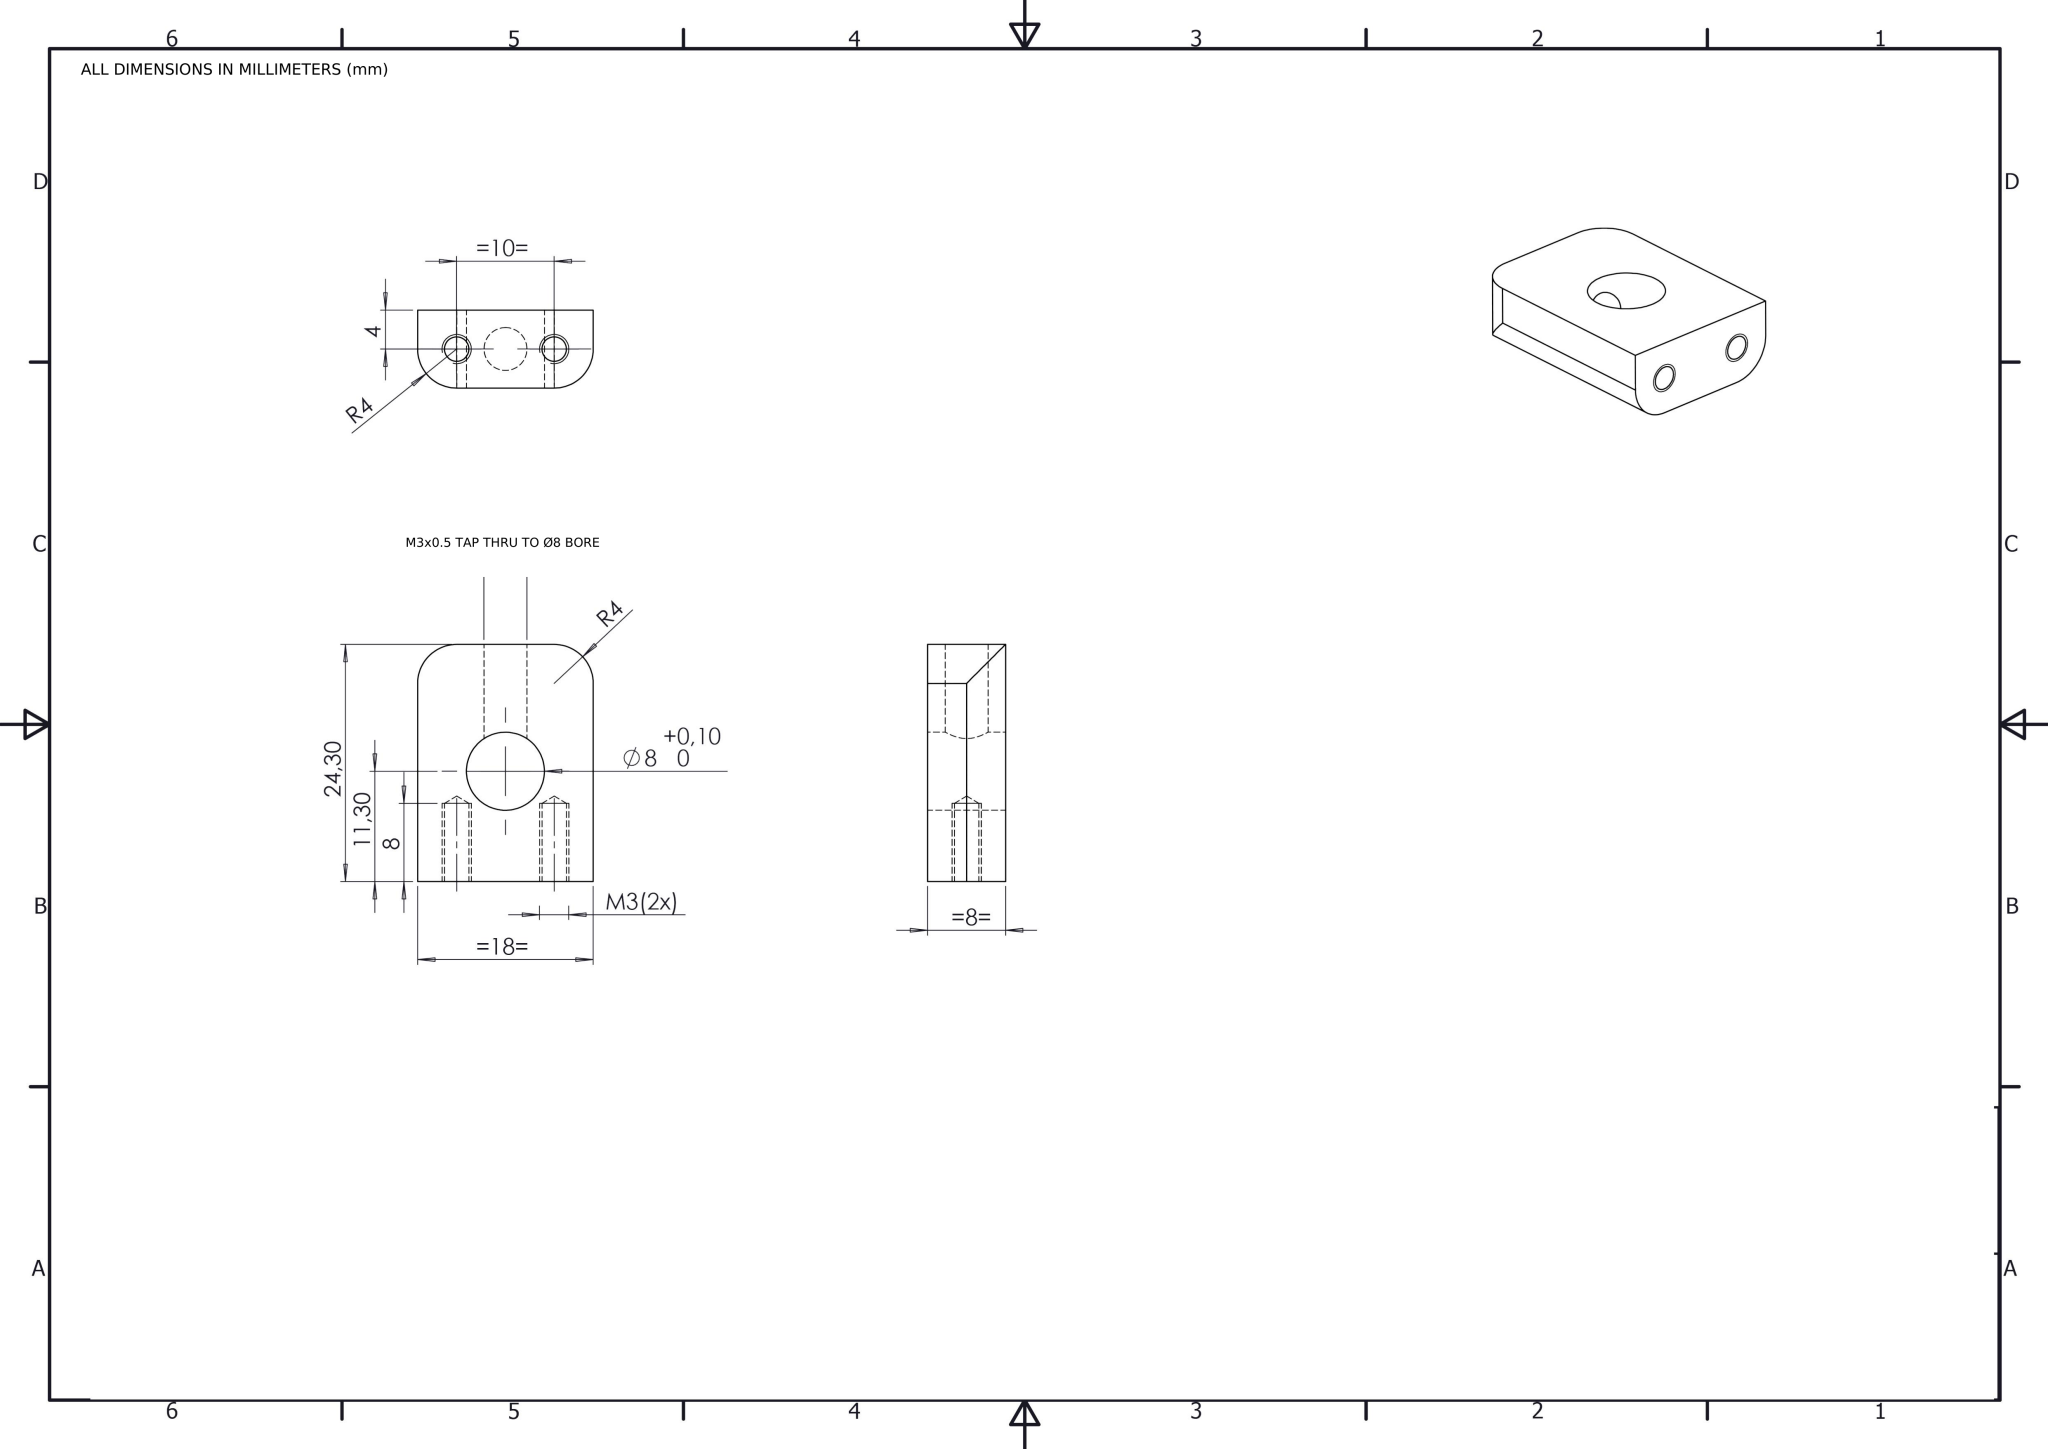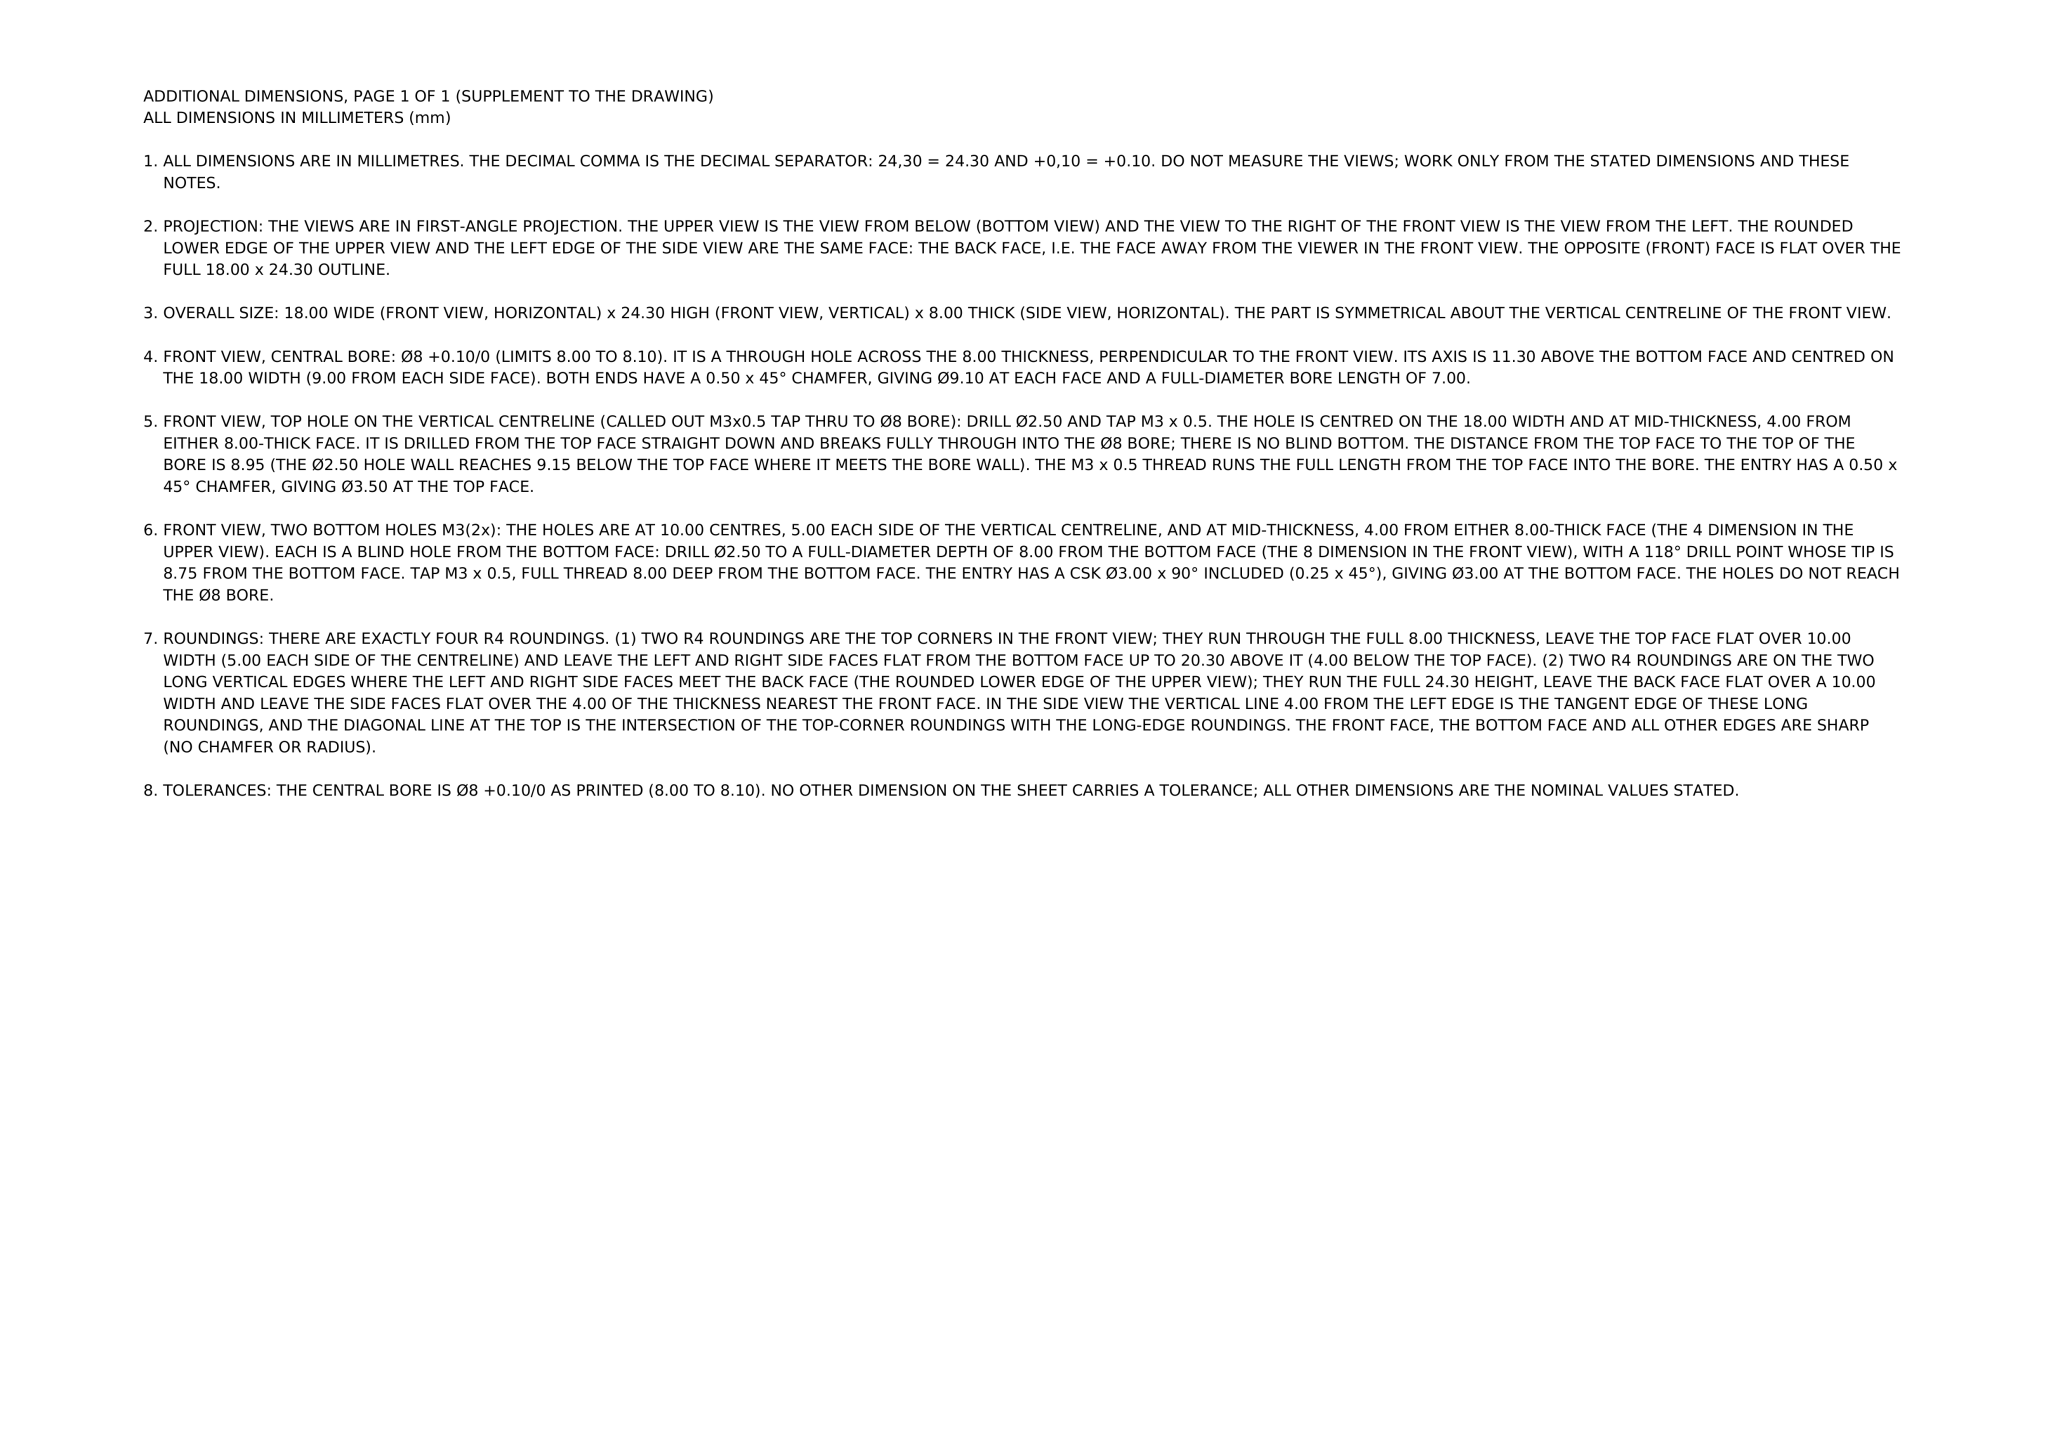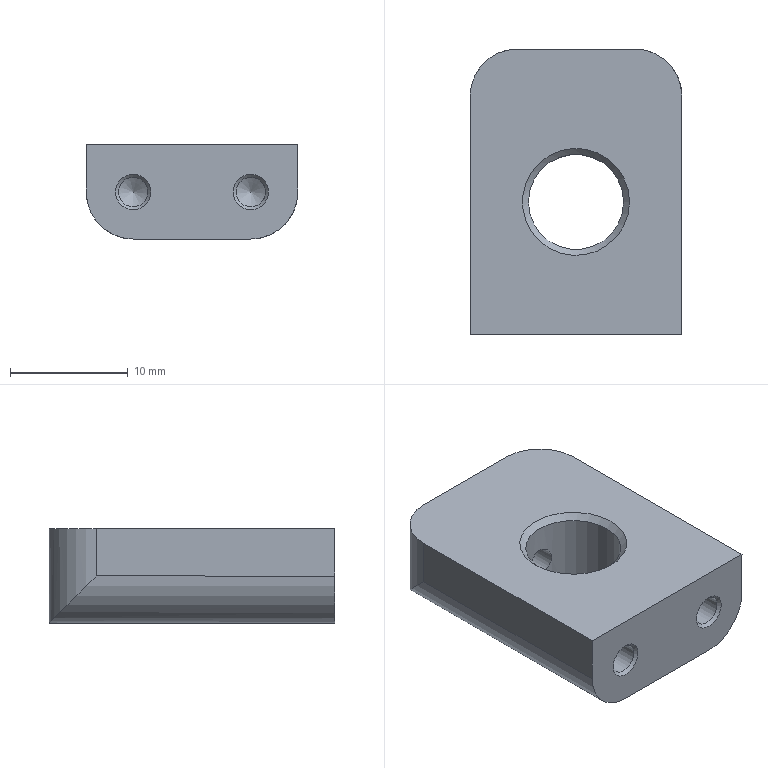Part | NX | mm | 1 solid | 21 faces | box 18 x 24.3 x 8 mm | volume 2744 mm3 | cylinder 8 | cone 7 | plane 6 | commonest cylinder face diameters 8 x4 2.5 x3 8.1 x1